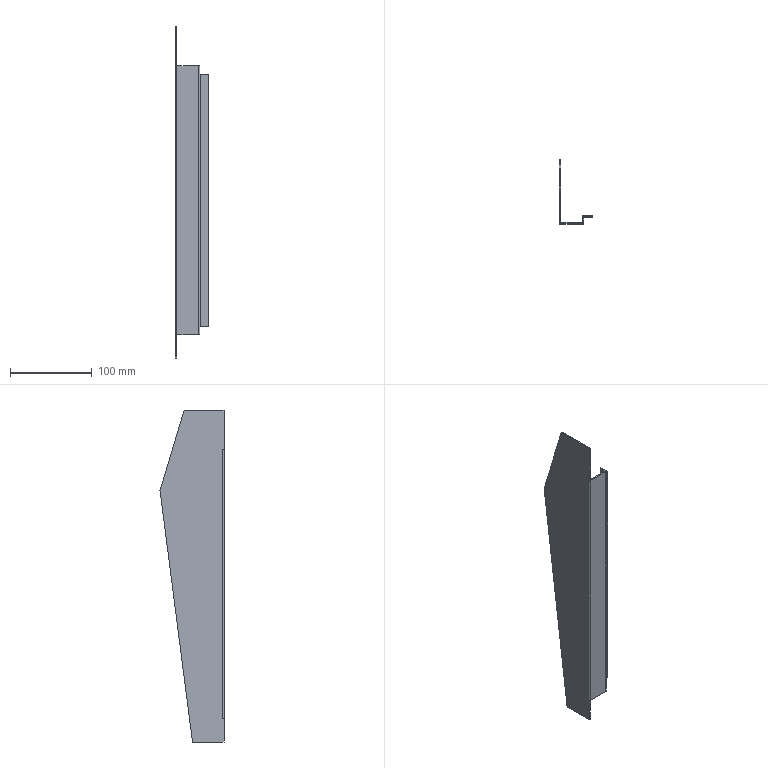Component | SolidWorks | TopCoverLeftSealingPlate-1 | 1 solid | 41 faces | volume 59166 mm3 | plane 35 | cylinder 6 | commonest cylinder face diameters 3.2 x3 0.2 x3